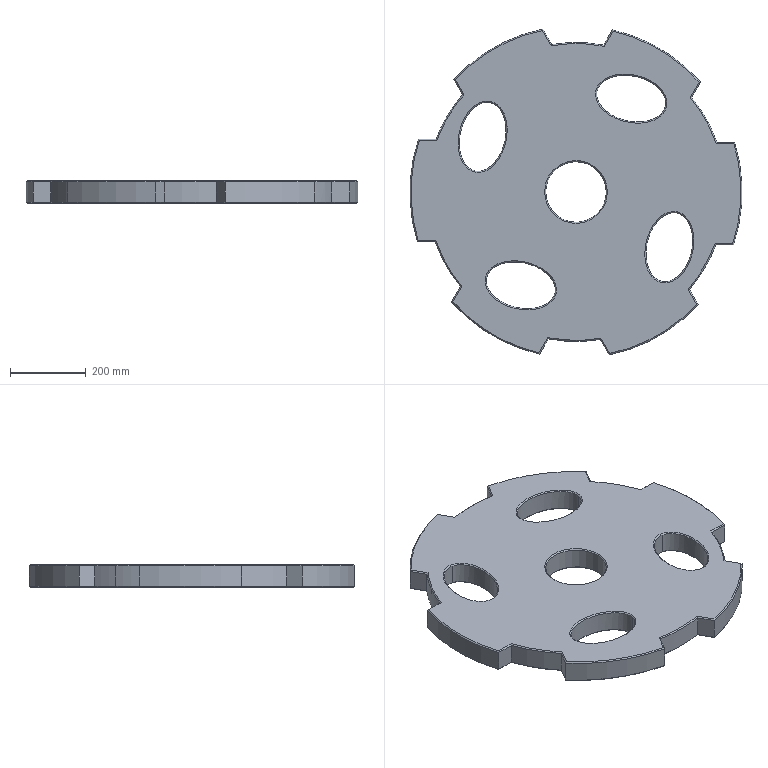Component | SolidWorks | WheelIndexingPlate-3 | 1 solid | 107 faces | volume 28323142 mm3 | plane 38 | cone 30 | spline 24 | cylinder 15 | commonest cylinder face diameters 790 x7 878 x6 160 x2 | material 45